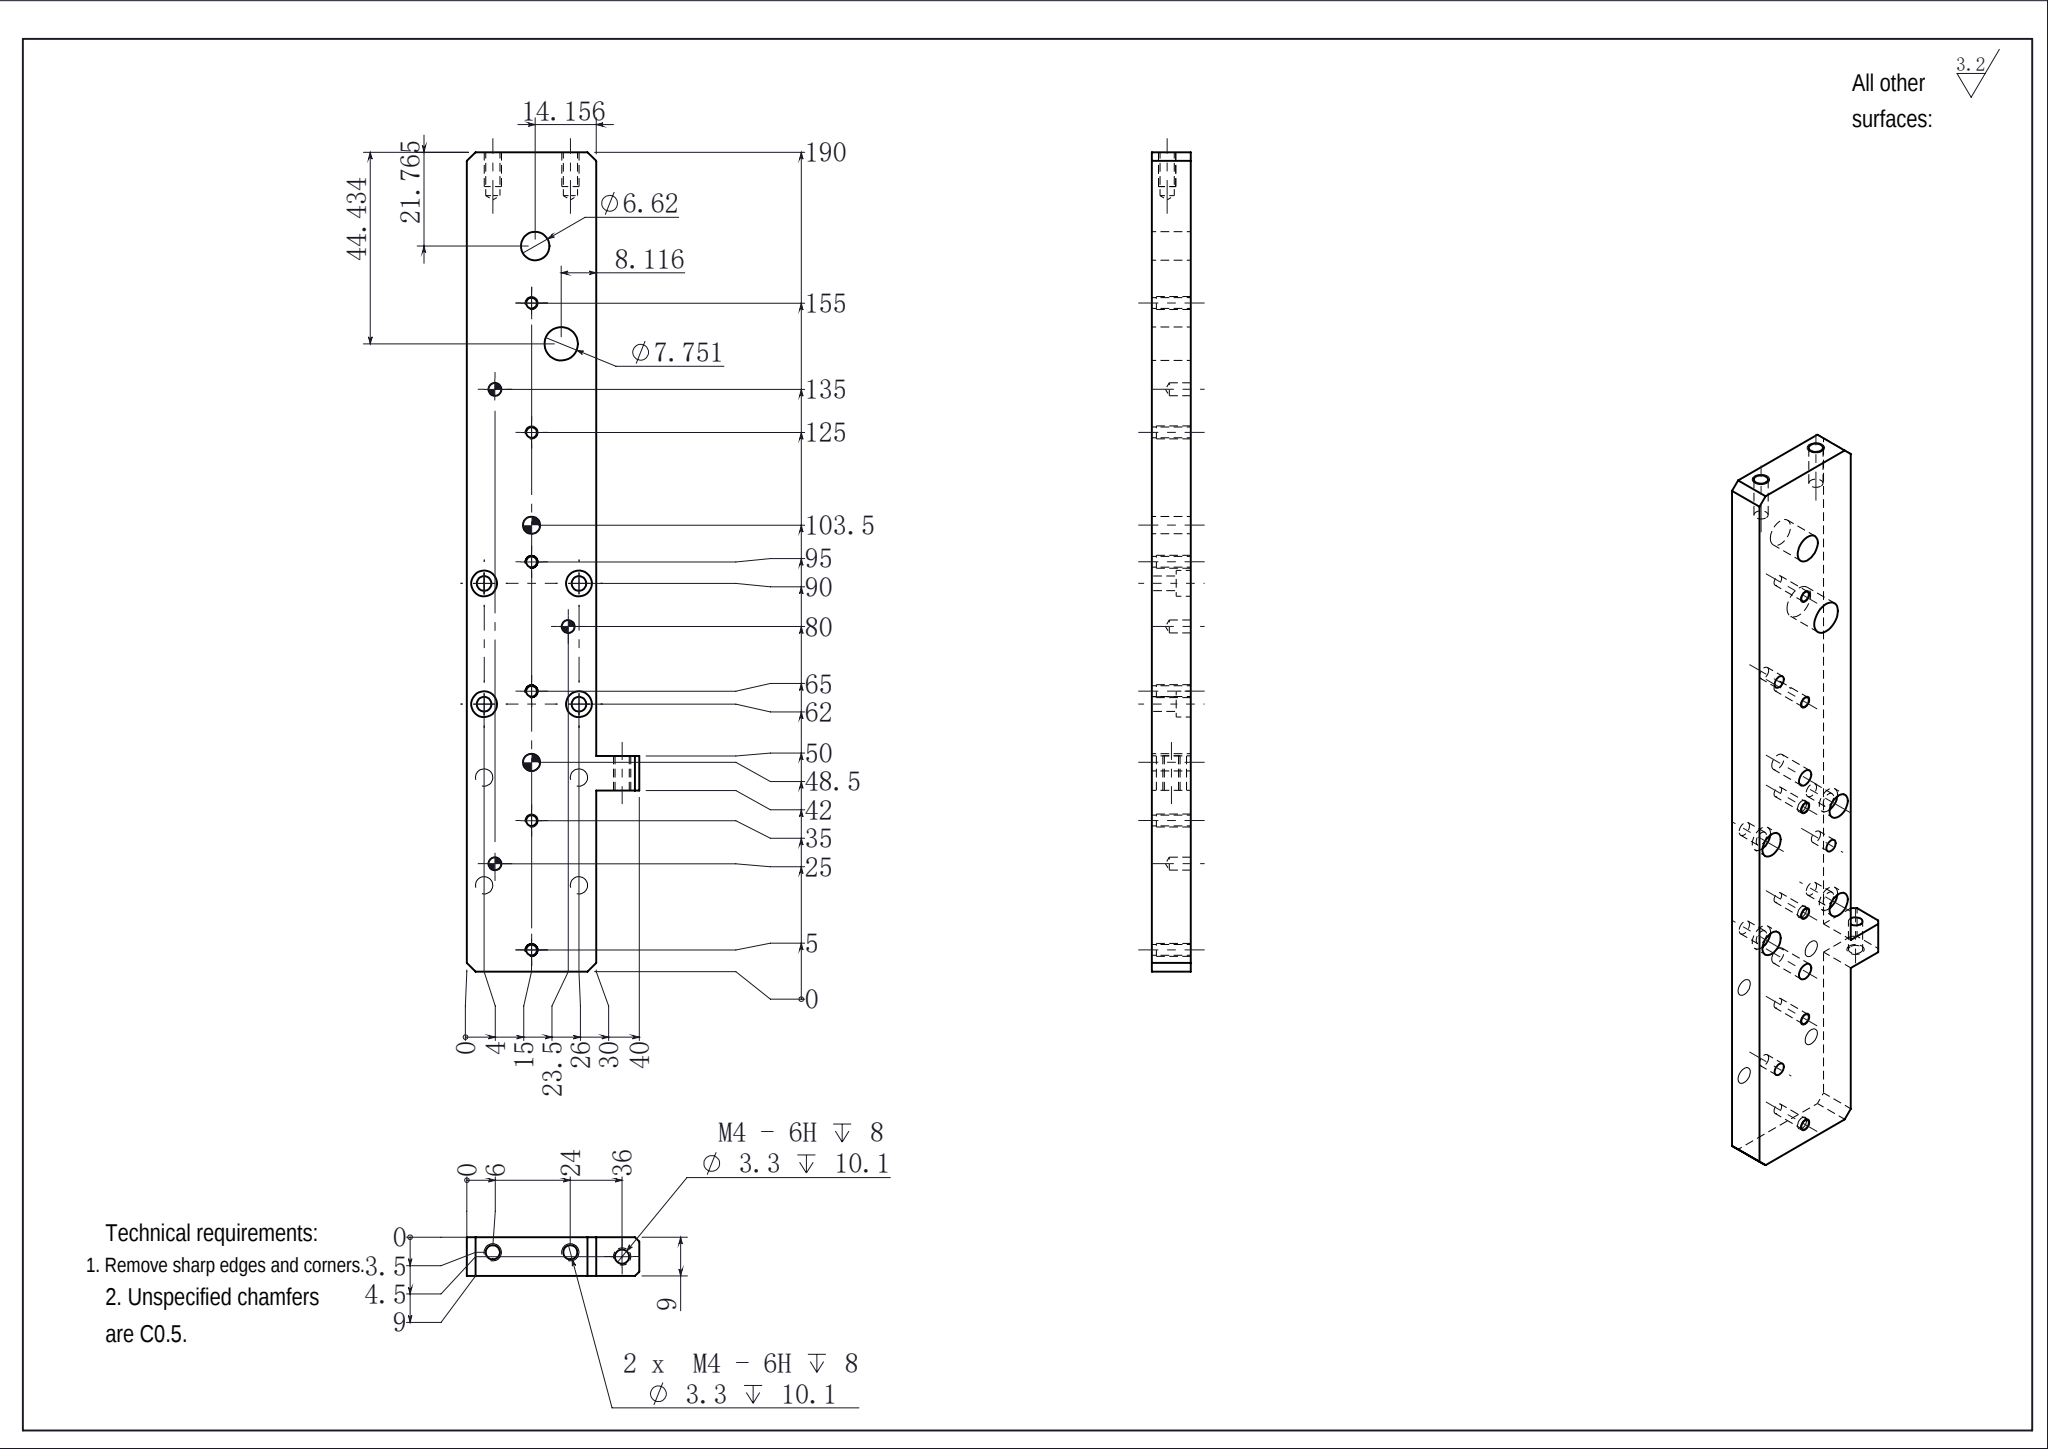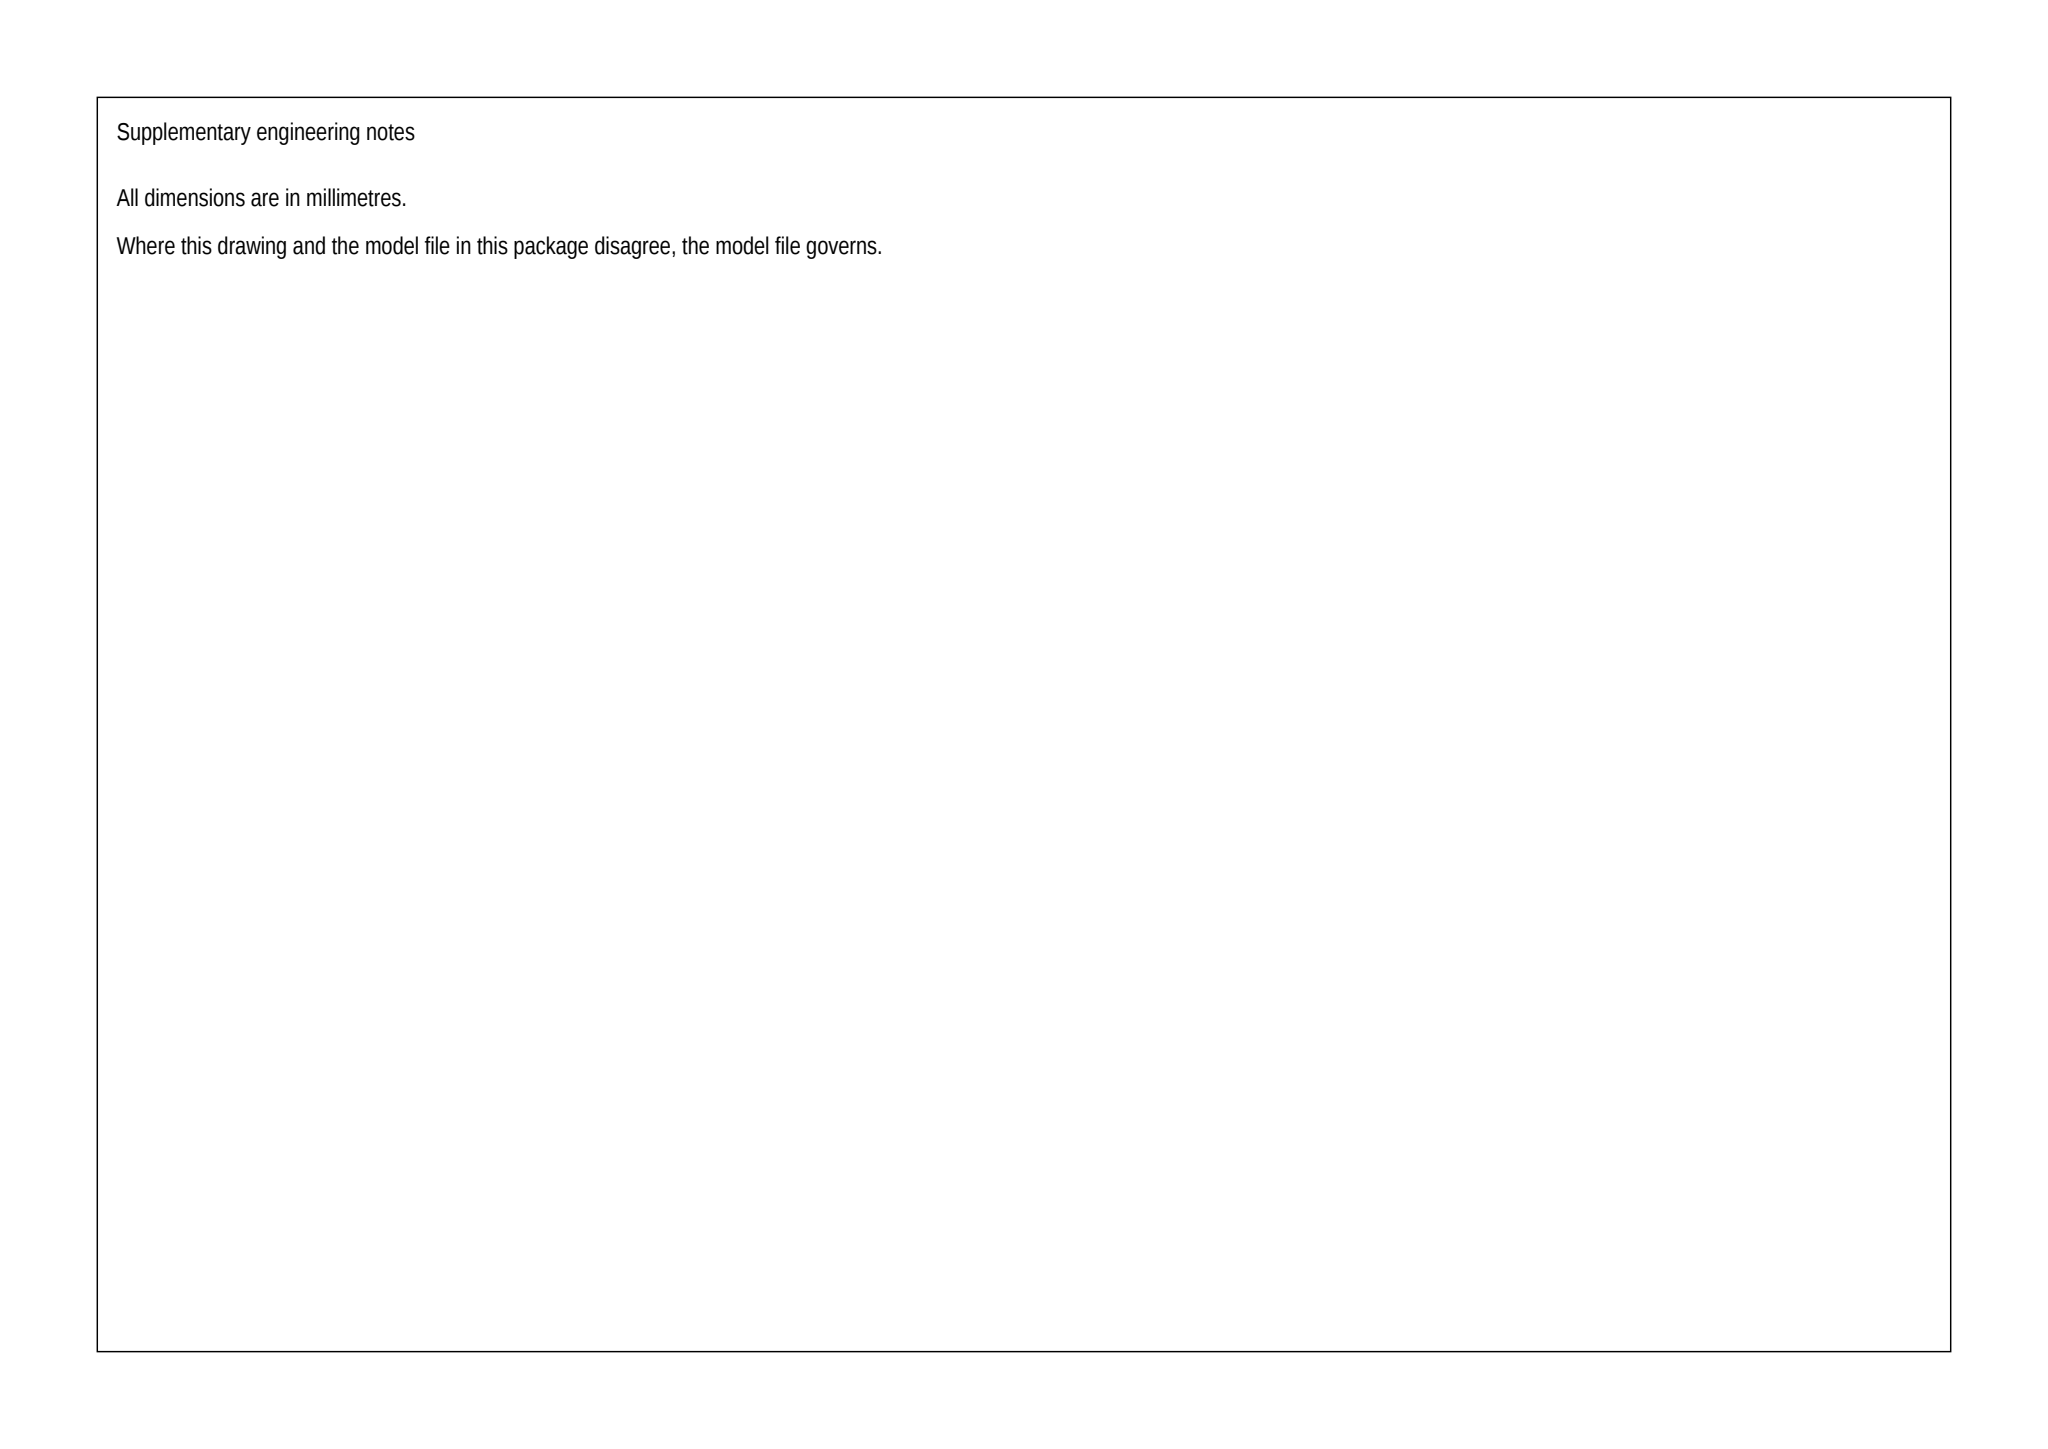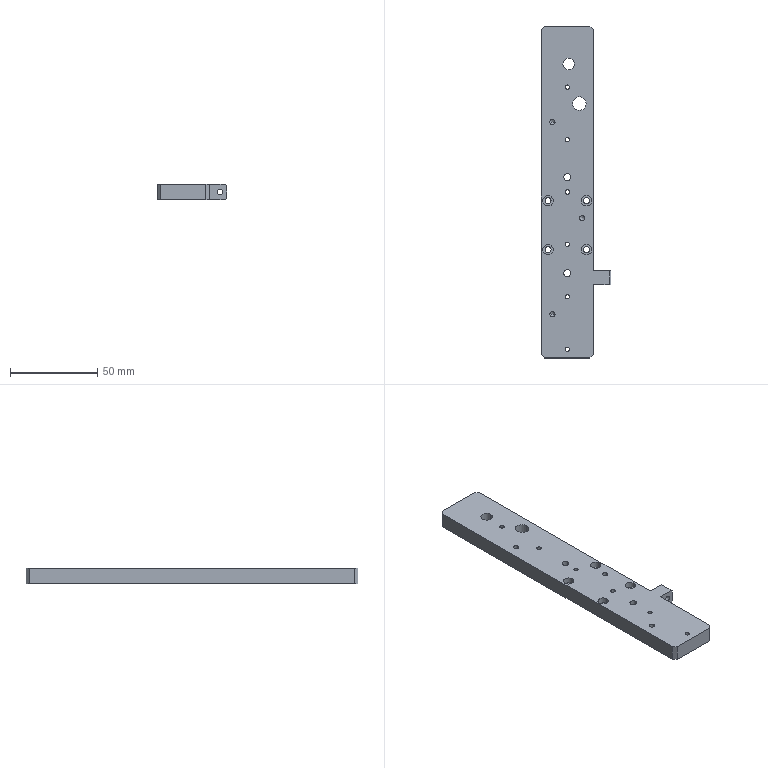Part | SolidWorks | mm | 1 solid | 78 faces | box 40 x 190 x 9 mm | volume 49767 mm3 | cylinder 48 | plane 20 | cone 10 | commonest cylinder face diameters 2.5 x12 6 x8 3.4 x8 3 x6 3.3 x6 4 x4 6.62 x2 7.751 x2
build123d program:
from build123d import *

# Parameters (mm, degrees)
SKETCH1_W                                          = 30
SKETCH1_H                                          = 190
BOSS_EXTRUDE1_DEPTH                                = 4.5
SKETCH2_W                                          = 9
SKETCH2_H                                          = 8
BOSS_EXTRUDE2_DEPTH                                = 10
M4_TAPPED_HOLE1_D                                  = 3.3
M4_TAPPED_HOLE1_DEPTH                              = 10.1
M4_TAPPED_HOLE1_TIP                                = 0.9914
M4_TAPPED_HOLE2_D                                  = 3.3
M4_TAPPED_HOLE2_DEPTH                              = 10.1
M4_TAPPED_HOLE2_TIP                                = 0.9914
CHAMFER1_SIZE                                      = 1
HOLE_SIZE_ACCORDING_TO_THE_TYPE_OF_HEX_D           = 3.4
HOLE_SIZE_ACCORDING_TO_THE_TYPE_OF_HEX_CBORE_D     = 6
HOLE_SIZE_ACCORDING_TO_THE_TYPE_OF_HEX_CBORE_DEPTH = 3.4
M3_TAPPED_HOLE2_D                                  = 2.5
M3_TAPPED_HOLE2_DEPTH                              = 10.5
M3_TAPPED_HOLE2_TIP                                = 0.7511
SIZE_MM_DOWEL_PIN_HOLE_2_D                         = 3
SIZE_MM_DOWEL_PIN_HOLE_2_DEPTH                     = 5
SIZE_MM_DOWEL_PIN_HOLE_2_TIP                       = 0.9013
SIZE_MM_DOWEL_PIN_HOLE_3_D                         = 4
CHAMFER2_SIZE                                      = 2
SKETCH25_R                                         = 3.31
SKETCH25_R_2                                       = 3.876
CUT_EXTRUDE2_DEPTH                                 = 80


with BuildPart() as part:
    # Sketch1 → Boss-Extrude1 (new, symmetric)
    with BuildSketch(Plane.XY):
        Rectangle(SKETCH1_W, SKETCH1_H)
    extrude(amount=BOSS_EXTRUDE1_DEPTH, both=True)

    # Sketch2 → Boss-Extrude2 (add)
    with BuildSketch(Plane(origin=(15, 0, 0), x_dir=(0, 0, -1), z_dir=(1, 0, 0))):
        with Locations((0, -49)):
            Rectangle(SKETCH2_W, SKETCH2_H)
    extrude(amount=BOSS_EXTRUDE2_DEPTH)

    # M4 Tapped Hole1
    with Locations(Plane(origin=(0, -53, 0), x_dir=(-1, 0, 0), z_dir=(0, -1, 0))):
        with Locations((-21, 0)):
            Hole(M4_TAPPED_HOLE1_D / 2, depth=M4_TAPPED_HOLE1_DEPTH)
            with Locations((0, 0, -(M4_TAPPED_HOLE1_DEPTH + M4_TAPPED_HOLE1_TIP / 2))):  # 118° drill point
                Cone(0, M4_TAPPED_HOLE1_D / 2, M4_TAPPED_HOLE1_TIP, mode=Mode.SUBTRACT)

    # M4 Tapped Hole2
    with Locations(Plane(origin=(0, 95, 0), x_dir=(1, 0, 0), z_dir=(0, 1, 0))):
        with Locations((-9, 1), (9, 1)):
            Hole(M4_TAPPED_HOLE2_D / 2, depth=M4_TAPPED_HOLE2_DEPTH)
            with Locations((0, 0, -(M4_TAPPED_HOLE2_DEPTH + M4_TAPPED_HOLE2_TIP / 2))):  # 118° drill point
                Cone(0, M4_TAPPED_HOLE2_D / 2, M4_TAPPED_HOLE2_TIP, mode=Mode.SUBTRACT)

    # Chamfer1
    chamfer1_edges = [part.edges().sort_by_distance(p)[0] for p in [
        (25, -49, -4.5),
        (25, -49, 4.5),
    ]]
    chamfer(chamfer1_edges, length=CHAMFER1_SIZE)

    # Hole size _according to_ the type of hex (through all)
    with Locations(Plane.XY.offset(4.5)):
        with Locations((-11, -5), (-11, -33), (11, -33), (11, -5)):
            CounterBoreHole(HOLE_SIZE_ACCORDING_TO_THE_TYPE_OF_HEX_D / 2, HOLE_SIZE_ACCORDING_TO_THE_TYPE_OF_HEX_CBORE_D / 2, HOLE_SIZE_ACCORDING_TO_THE_TYPE_OF_HEX_CBORE_DEPTH)

    # M3 Tapped Hole2
    with Locations(Plane.XY.offset(4.5)):
        with Locations((0, 60), (0, 30), (0, 0), (0, -30), (0, -60), (0, -90)):
            Hole(M3_TAPPED_HOLE2_D / 2, depth=M3_TAPPED_HOLE2_DEPTH)
            with Locations((0, 0, -(M3_TAPPED_HOLE2_DEPTH + M3_TAPPED_HOLE2_TIP / 2))):  # 118° drill point
                Cone(0, M3_TAPPED_HOLE2_D / 2, M3_TAPPED_HOLE2_TIP, mode=Mode.SUBTRACT)

    # Size mm Dowel Pin Hole 2
    with Locations(Plane.XY.offset(4.5)):
        with Locations((-8.5, 40), (-8.5, -70), (8.5, -15)):
            Hole(SIZE_MM_DOWEL_PIN_HOLE_2_D / 2, depth=SIZE_MM_DOWEL_PIN_HOLE_2_DEPTH)
            with Locations((0, 0, -(SIZE_MM_DOWEL_PIN_HOLE_2_DEPTH + SIZE_MM_DOWEL_PIN_HOLE_2_TIP / 2))):  # 118° drill point
                Cone(0, SIZE_MM_DOWEL_PIN_HOLE_2_D / 2, SIZE_MM_DOWEL_PIN_HOLE_2_TIP, mode=Mode.SUBTRACT)

    # Size mm Dowel Pin Hole 3 (through all)
    with Locations(Plane.XY.offset(4.5)):
        with Locations((0, 8.5), (0, -46.5)):
            Hole(SIZE_MM_DOWEL_PIN_HOLE_3_D / 2)

    # Chamfer2
    chamfer2_edges = [part.edges().sort_by_distance(p)[0] for p in [
        (15, -95, 0),
        (-15, -95, 0),
        (15, 95, 0),
        (-15, 95, 0),
    ]]
    chamfer(chamfer2_edges, length=CHAMFER2_SIZE)

    # Sketch25 → Cut-Extrude2 (cut)
    with BuildSketch(Plane.XY.offset(4.5)):
        with Locations((0.8438, 73.235)):
            Circle(SKETCH25_R)
        with Locations((6.884, 50.566)):
            Circle(SKETCH25_R_2)
    extrude(amount=-CUT_EXTRUDE2_DEPTH, mode=Mode.SUBTRACT)


solid = part.part